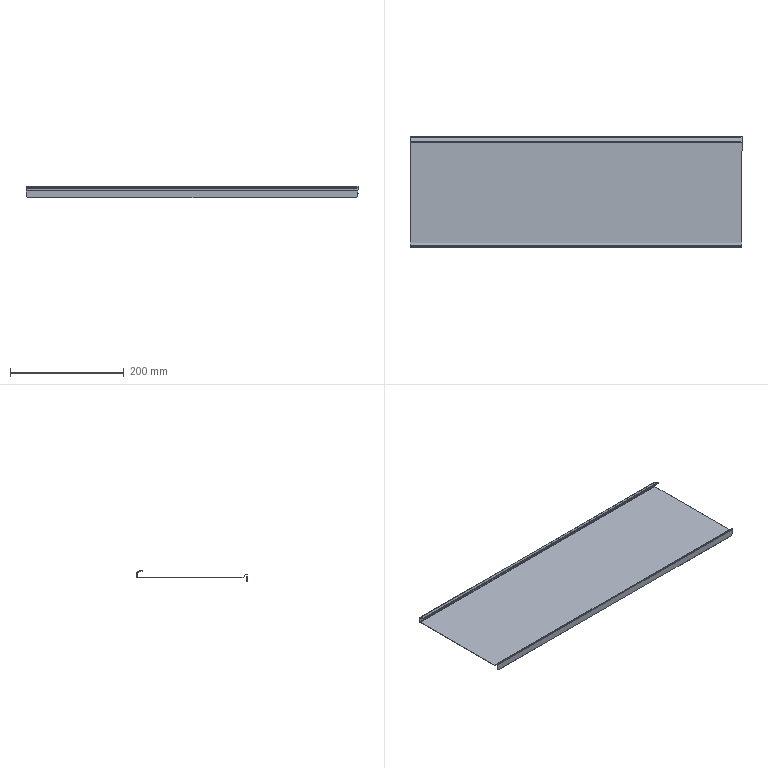Component | SolidWorks | PC-CAJ-P08-1_PC-CAJ-P18-1_PM-CAJ-P59-1 | 1 solid | 50 faces | volume 95648 mm3 | plane 38 | cylinder 12 | commonest cylinder face diameters 2.4 x5 1 x4 0.2 x2 1.6 x1 | material Plain Carbon Steel